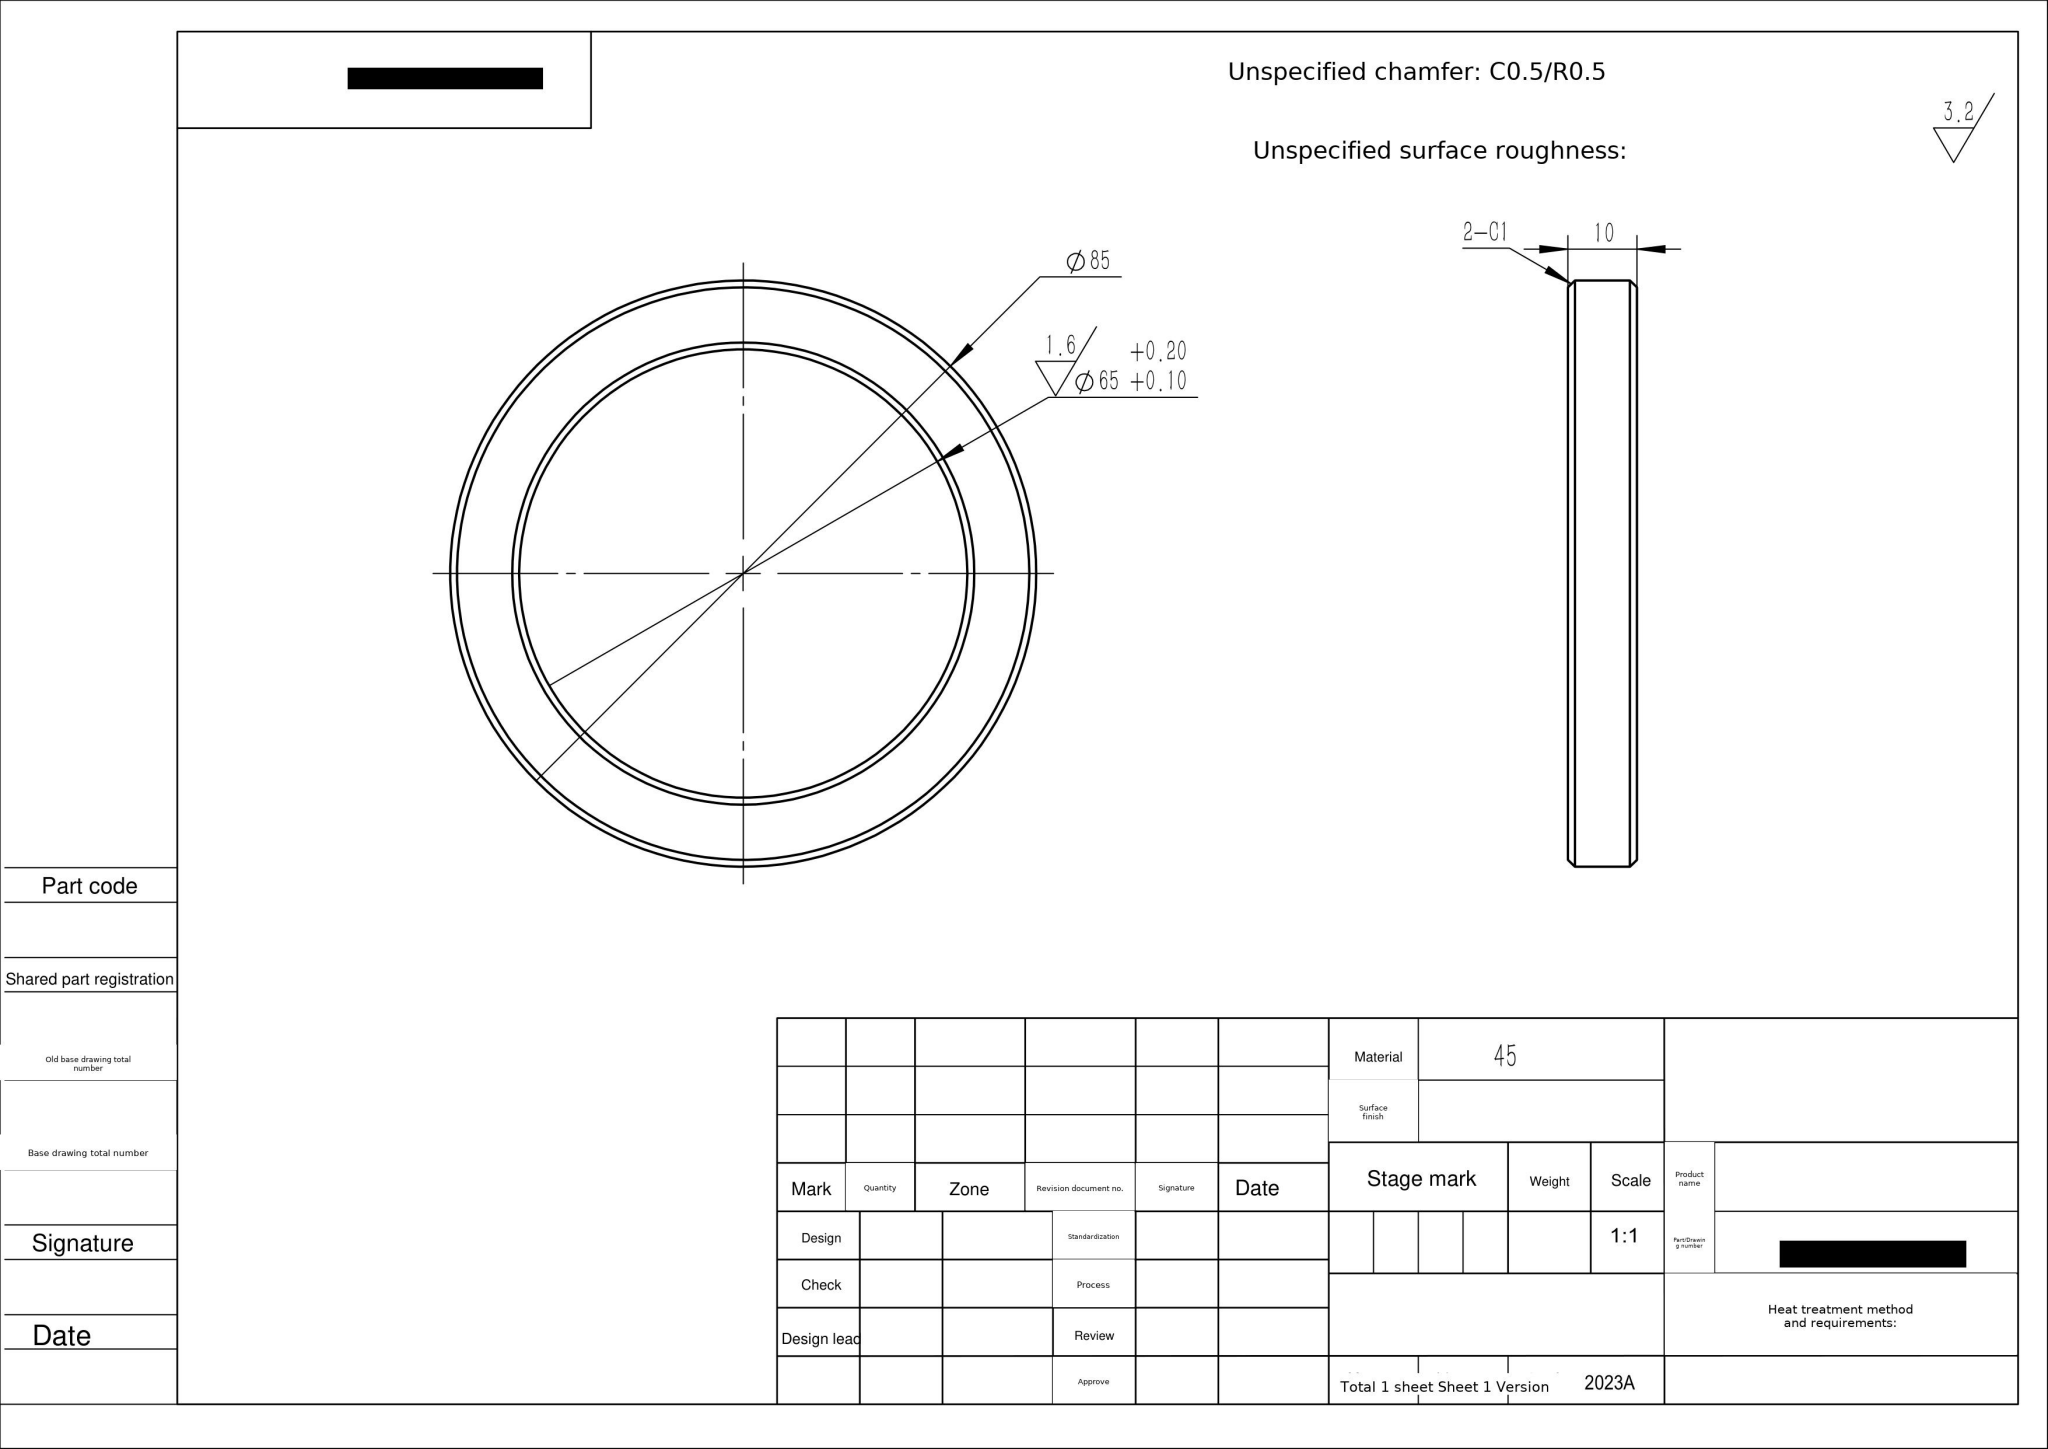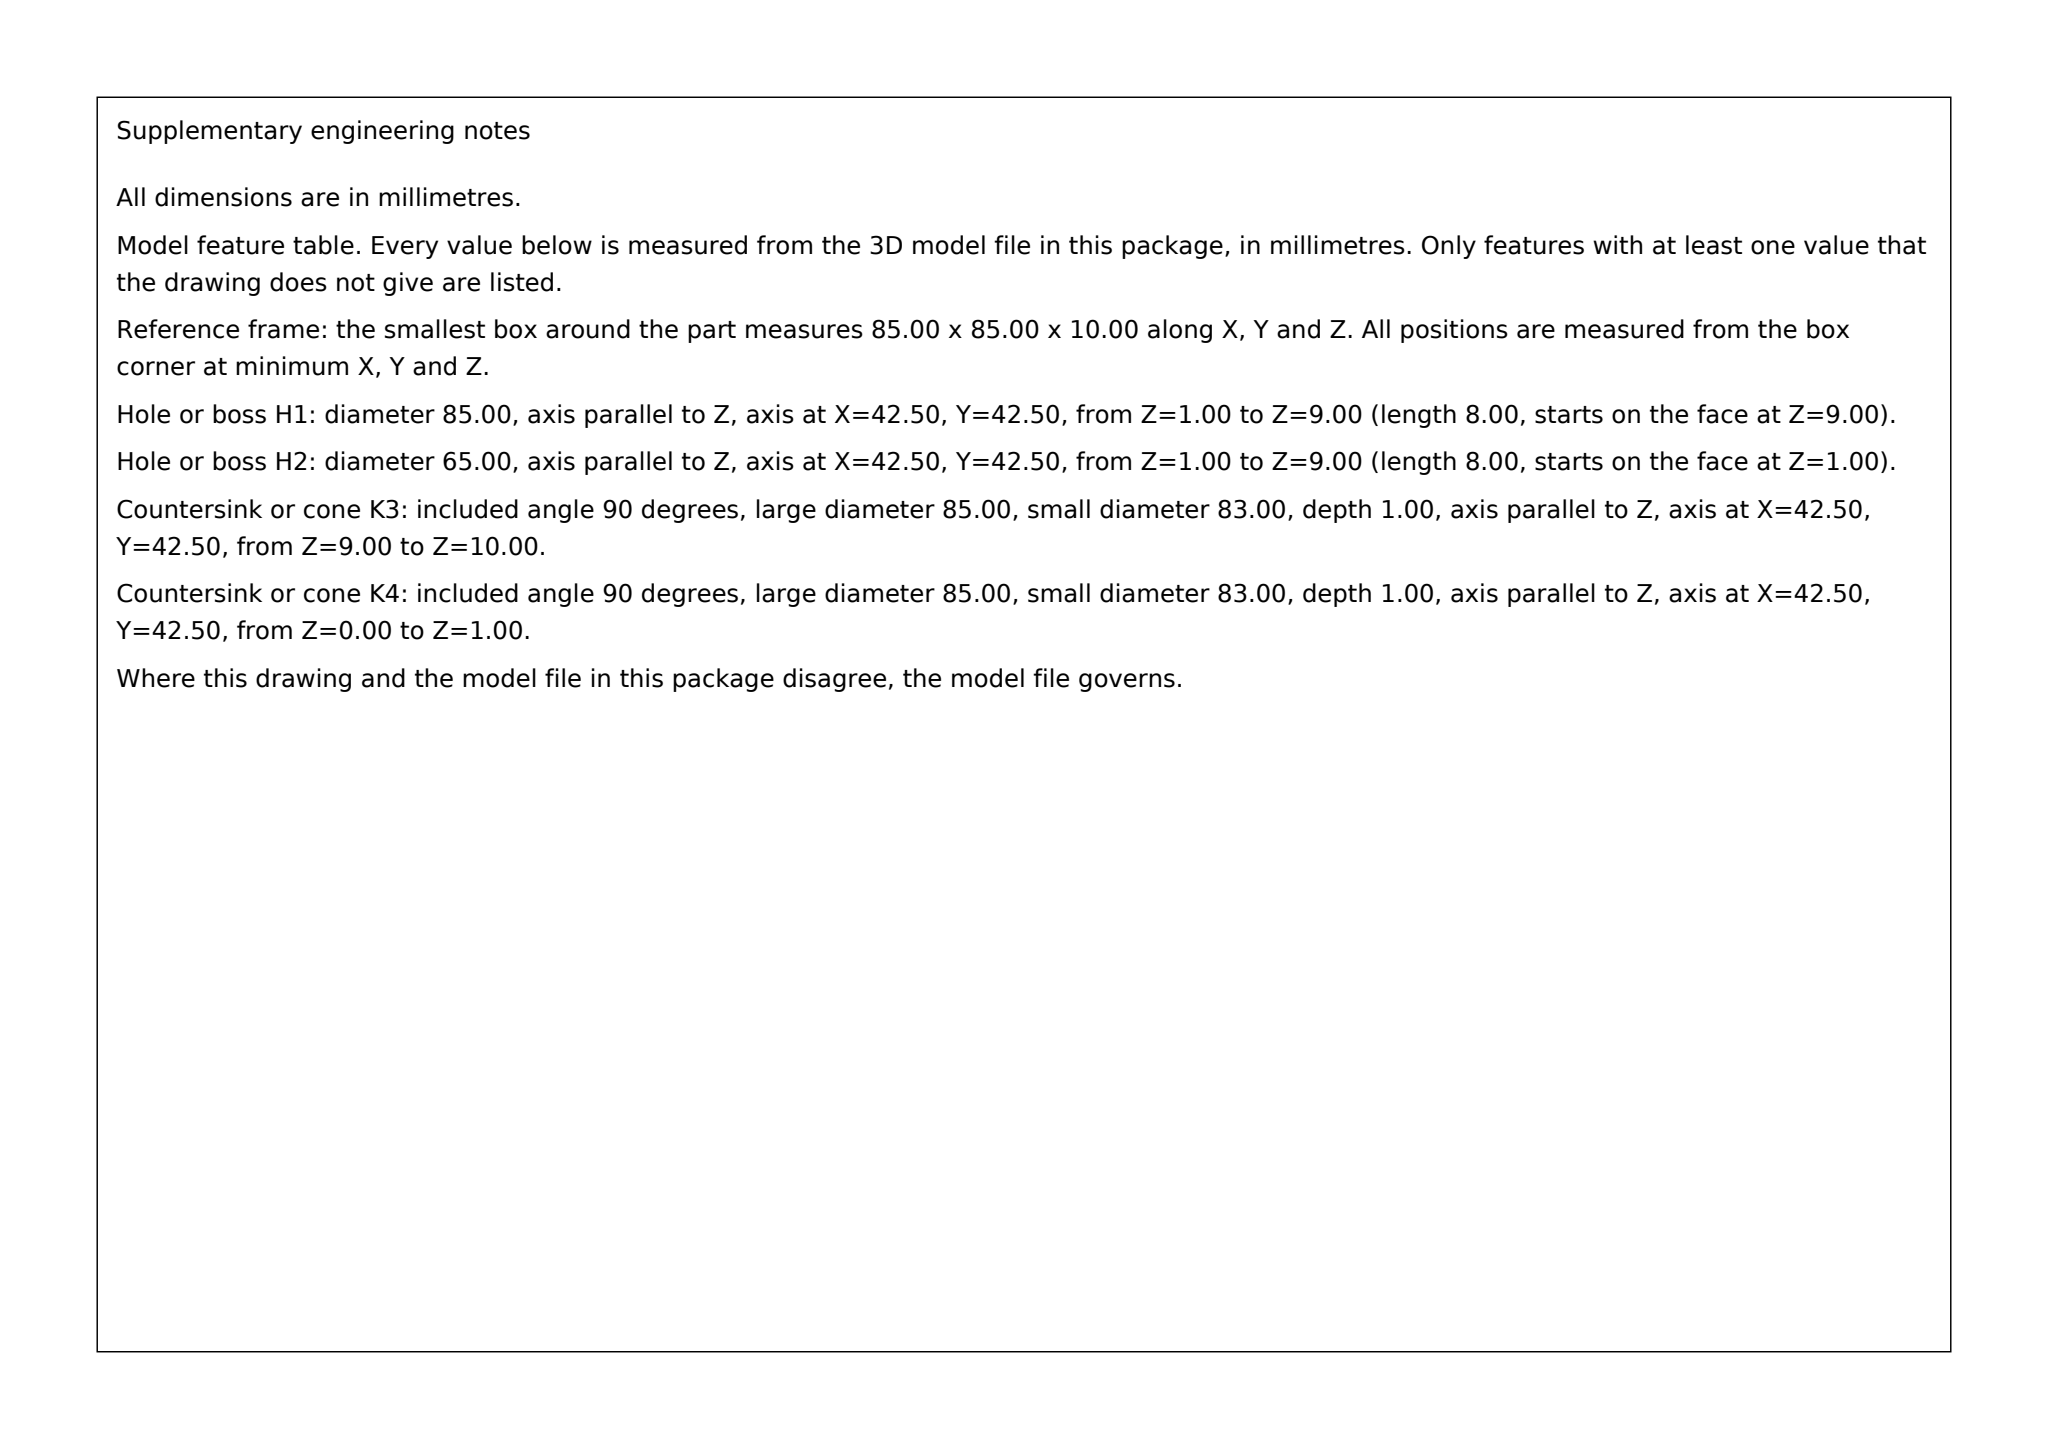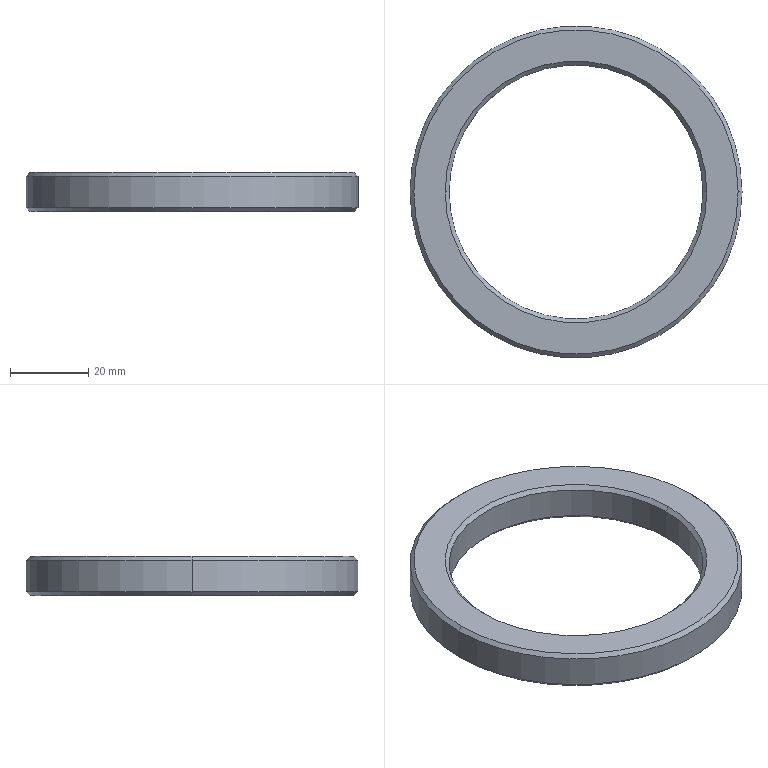Part | SolidWorks | mm | material 45 | 1 solid | 14 faces | box 85 x 85 x 10 mm | volume 23091 mm3 | cone 8 | cylinder 4 | plane 2 | commonest cylinder face diameters 65 x2 85 x2
build123d program:
from build123d import *

# Parameters (mm, degrees)
SKETCH1_R           = 42.5
SKETCH1_R_2         = 32.5
BOSS_EXTRUDE1_DEPTH = 10
CHAMFER1_SIZE       = 1


with BuildPart() as part:
    # Sketch1 → Boss-Extrude1 (new body)
    with BuildSketch(Plane.XY):
        Circle(SKETCH1_R)
        Circle(SKETCH1_R_2, mode=Mode.SUBTRACT)
    extrude(amount=BOSS_EXTRUDE1_DEPTH)

    # Chamfer1
    chamfer1_edges = [part.edges().sort_by_distance(p)[0] for p in [
        (-42.5, 0, 0),
        (-42.5, 0, 10),
        (-32.5, 0, 0),
        (-32.5, 0, 10),
    ]]
    chamfer(chamfer1_edges, length=CHAMFER1_SIZE)


solid = part.part
STEP:
#1=CARTESIAN_POINT('',(41.5,0.,10.));
#2=VERTEX_POINT('',#1);
#3=CARTESIAN_POINT('',(-41.5,0.,10.));
#4=VERTEX_POINT('',#3);
#5=CARTESIAN_POINT('',(0.,0.,10.));
#6=DIRECTION('',(0.,0.,1.));
#7=DIRECTION('',(1.,0.,0.));
#8=AXIS2_PLACEMENT_3D('',#5,#6,#7);
#9=CIRCLE('',#8,41.5);
#10=EDGE_CURVE('',#2,#4,#9,.T.);
#11=ORIENTED_EDGE('',*,*,#10,.F.);
#12=CARTESIAN_POINT('',(42.5,0.,9.));
#13=VERTEX_POINT('',#12);
#14=CARTESIAN_POINT('',(41.5,0.,10.));
#15=DIRECTION('',(0.7071,0.,-0.7071));
#16=VECTOR('',#15,1000.);
#17=LINE('',#14,#16);
#18=EDGE_CURVE('',#2,#13,#17,.T.);
#19=ORIENTED_EDGE('',*,*,#18,.T.);
#20=CARTESIAN_POINT('',(-42.5,0.,9.));
#21=VERTEX_POINT('',#20);
#22=CARTESIAN_POINT('',(0.,0.,9.));
#23=DIRECTION('',(0.,0.,-1.));
#24=DIRECTION('',(1.,0.,0.));
#25=AXIS2_PLACEMENT_3D('',#22,#23,#24);
#26=CIRCLE('',#25,42.5);
#27=EDGE_CURVE('',#21,#13,#26,.T.);
#28=ORIENTED_EDGE('',*,*,#27,.F.);
#29=CARTESIAN_POINT('',(-41.5,0.,10.));
#30=DIRECTION('',(-0.7071,0.,-0.7071));
#31=VECTOR('',#30,1000.);
#32=LINE('',#29,#31);
#33=EDGE_CURVE('',#4,#21,#32,.T.);
#34=ORIENTED_EDGE('',*,*,#33,.F.);
#35=EDGE_LOOP('',(#11,#19,#28,#34));
#36=FACE_OUTER_BOUND('',#35,.T.);
#37=CARTESIAN_POINT('',(0.,0.,10.));
#38=DIRECTION('',(0.,0.,-1.));
#39=DIRECTION('',(-1.,0.,0.));
#40=AXIS2_PLACEMENT_3D('',#37,#38,#39);
#41=CONICAL_SURFACE('',#40,41.5,0.7854);
#42=ADVANCED_FACE('',(#36),#41,.T.);
#43=CARTESIAN_POINT('',(-41.5,0.,0.));
#44=VERTEX_POINT('',#43);
#45=CARTESIAN_POINT('',(41.5,0.,0.));
#46=VERTEX_POINT('',#45);
#47=CARTESIAN_POINT('',(0.,0.,0.));
#48=DIRECTION('',(0.,0.,-1.));
#49=DIRECTION('',(1.,0.,0.));
#50=AXIS2_PLACEMENT_3D('',#47,#48,#49);
#51=CIRCLE('',#50,41.5);
#52=EDGE_CURVE('',#44,#46,#51,.T.);
#53=ORIENTED_EDGE('',*,*,#52,.F.);
#54=CARTESIAN_POINT('',(-42.5,0.,1.));
#55=VERTEX_POINT('',#54);
#56=CARTESIAN_POINT('',(-42.5,0.,1.));
#57=DIRECTION('',(-0.7071,0.,0.7071));
#58=VECTOR('',#57,1000.);
#59=LINE('',#56,#58);
#60=EDGE_CURVE('',#44,#55,#59,.T.);
#61=ORIENTED_EDGE('',*,*,#60,.T.);
#62=CARTESIAN_POINT('',(42.5,0.,1.));
#63=VERTEX_POINT('',#62);
#64=CARTESIAN_POINT('',(0.,0.,1.));
#65=DIRECTION('',(0.,0.,1.));
#66=DIRECTION('',(1.,0.,0.));
#67=AXIS2_PLACEMENT_3D('',#64,#65,#66);
#68=CIRCLE('',#67,42.5);
#69=EDGE_CURVE('',#63,#55,#68,.T.);
#70=ORIENTED_EDGE('',*,*,#69,.F.);
#71=CARTESIAN_POINT('',(42.5,0.,1.));
#72=DIRECTION('',(0.7071,0.,0.7071));
#73=VECTOR('',#72,1000.);
#74=LINE('',#71,#73);
#75=EDGE_CURVE('',#46,#63,#74,.T.);
#76=ORIENTED_EDGE('',*,*,#75,.F.);
#77=EDGE_LOOP('',(#53,#61,#70,#76));
#78=FACE_OUTER_BOUND('',#77,.T.);
#79=CARTESIAN_POINT('',(0.,0.,1.));
#80=DIRECTION('',(0.,0.,1.));
#81=DIRECTION('',(1.,0.,0.));
#82=AXIS2_PLACEMENT_3D('',#79,#80,#81);
#83=CONICAL_SURFACE('',#82,42.5,0.7854);
#84=ADVANCED_FACE('',(#78),#83,.T.);
#85=CARTESIAN_POINT('',(32.5,0.,1.));
#86=VERTEX_POINT('',#85);
#87=CARTESIAN_POINT('',(-32.5,0.,1.));
#88=VERTEX_POINT('',#87);
#89=CARTESIAN_POINT('',(0.,0.,1.));
#90=DIRECTION('',(0.,0.,-1.));
#91=DIRECTION('',(1.,0.,0.));
#92=AXIS2_PLACEMENT_3D('',#89,#90,#91);
#93=CIRCLE('',#92,32.5);
#94=EDGE_CURVE('',#86,#88,#93,.T.);
#95=ORIENTED_EDGE('',*,*,#94,.F.);
#96=CARTESIAN_POINT('',(33.5,0.,0.));
#97=VERTEX_POINT('',#96);
#98=CARTESIAN_POINT('',(33.5,0.,0.));
#99=DIRECTION('',(0.7071,0.,-0.7071));
#100=VECTOR('',#99,1000.);
#101=LINE('',#98,#100);
#102=EDGE_CURVE('',#86,#97,#101,.T.);
#103=ORIENTED_EDGE('',*,*,#102,.T.);
#104=CARTESIAN_POINT('',(-33.5,0.,0.));
#105=VERTEX_POINT('',#104);
#106=CARTESIAN_POINT('',(0.,0.,0.));
#107=DIRECTION('',(0.,0.,1.));
#108=DIRECTION('',(1.,0.,0.));
#109=AXIS2_PLACEMENT_3D('',#106,#107,#108);
#110=CIRCLE('',#109,33.5);
#111=EDGE_CURVE('',#105,#97,#110,.T.);
#112=ORIENTED_EDGE('',*,*,#111,.F.);
#113=CARTESIAN_POINT('',(-33.5,0.,0.));
#114=DIRECTION('',(-0.7071,0.,-0.7071));
#115=VECTOR('',#114,1000.);
#116=LINE('',#113,#115);
#117=EDGE_CURVE('',#88,#105,#116,.T.);
#118=ORIENTED_EDGE('',*,*,#117,.F.);
#119=EDGE_LOOP('',(#95,#103,#112,#118));
#120=FACE_OUTER_BOUND('',#119,.T.);
#121=CARTESIAN_POINT('',(0.,0.,0.));
#122=DIRECTION('',(0.,0.,-1.));
#123=DIRECTION('',(-1.,0.,0.));
#124=AXIS2_PLACEMENT_3D('',#121,#122,#123);
#125=CONICAL_SURFACE('',#124,33.5,0.7854);
#126=ADVANCED_FACE('',(#120),#125,.F.);
#127=CARTESIAN_POINT('',(-32.5,0.,9.));
#128=VERTEX_POINT('',#127);
#129=CARTESIAN_POINT('',(32.5,0.,9.));
#130=VERTEX_POINT('',#129);
#131=CARTESIAN_POINT('',(0.,0.,9.));
#132=DIRECTION('',(0.,0.,1.));
#133=DIRECTION('',(1.,0.,0.));
#134=AXIS2_PLACEMENT_3D('',#131,#132,#133);
#135=CIRCLE('',#134,32.5);
#136=EDGE_CURVE('',#128,#130,#135,.T.);
#137=ORIENTED_EDGE('',*,*,#136,.F.);
#138=CARTESIAN_POINT('',(-33.5,0.,10.));
#139=VERTEX_POINT('',#138);
#140=CARTESIAN_POINT('',(-32.5,0.,9.));
#141=DIRECTION('',(-0.7071,0.,0.7071));
#142=VECTOR('',#141,1000.);
#143=LINE('',#140,#142);
#144=EDGE_CURVE('',#128,#139,#143,.T.);
#145=ORIENTED_EDGE('',*,*,#144,.T.);
#146=CARTESIAN_POINT('',(33.5,0.,10.));
#147=VERTEX_POINT('',#146);
#148=CARTESIAN_POINT('',(0.,0.,10.));
#149=DIRECTION('',(0.,0.,-1.));
#150=DIRECTION('',(1.,0.,0.));
#151=AXIS2_PLACEMENT_3D('',#148,#149,#150);
#152=CIRCLE('',#151,33.5);
#153=EDGE_CURVE('',#147,#139,#152,.T.);
#154=ORIENTED_EDGE('',*,*,#153,.F.);
#155=CARTESIAN_POINT('',(32.5,0.,9.));
#156=DIRECTION('',(0.7071,0.,0.7071));
#157=VECTOR('',#156,1000.);
#158=LINE('',#155,#157);
#159=EDGE_CURVE('',#130,#147,#158,.T.);
#160=ORIENTED_EDGE('',*,*,#159,.F.);
#161=EDGE_LOOP('',(#137,#145,#154,#160));
#162=FACE_OUTER_BOUND('',#161,.T.);
#163=CARTESIAN_POINT('',(0.,0.,9.));
#164=DIRECTION('',(0.,0.,1.));
#165=DIRECTION('',(1.,0.,0.));
#166=AXIS2_PLACEMENT_3D('',#163,#164,#165);
#167=CONICAL_SURFACE('',#166,32.5,0.7854);
#168=ADVANCED_FACE('',(#162),#167,.F.);
#169=ORIENTED_EDGE('',*,*,#136,.T.);
#170=CARTESIAN_POINT('',(32.5,0.,10.));
#171=DIRECTION('',(0.,0.,-1.));
#172=VECTOR('',#171,1000.);
#173=LINE('',#170,#172);
#174=EDGE_CURVE('',#130,#86,#173,.T.);
#175=ORIENTED_EDGE('',*,*,#174,.T.);
#176=ORIENTED_EDGE('',*,*,#94,.T.);
#177=CARTESIAN_POINT('',(-32.5,0.,10.));
#178=DIRECTION('',(0.,0.,-1.));
#179=VECTOR('',#178,1000.);
#180=LINE('',#177,#179);
#181=EDGE_CURVE('',#128,#88,#180,.T.);
#182=ORIENTED_EDGE('',*,*,#181,.F.);
#183=EDGE_LOOP('',(#169,#175,#176,#182));
#184=FACE_OUTER_BOUND('',#183,.T.);
#185=CARTESIAN_POINT('',(0.,0.,10.));
#186=DIRECTION('',(0.,0.,-1.));
#187=DIRECTION('',(-1.,0.,0.));
#188=AXIS2_PLACEMENT_3D('',#185,#186,#187);
#189=CYLINDRICAL_SURFACE('',#188,32.5);
#190=ADVANCED_FACE('',(#184),#189,.F.);
#191=ORIENTED_EDGE('',*,*,#27,.T.);
#192=CARTESIAN_POINT('',(42.5,0.,10.));
#193=DIRECTION('',(0.,0.,-1.));
#194=VECTOR('',#193,1000.);
#195=LINE('',#192,#194);
#196=EDGE_CURVE('',#13,#63,#195,.T.);
#197=ORIENTED_EDGE('',*,*,#196,.T.);
#198=ORIENTED_EDGE('',*,*,#69,.T.);
#199=CARTESIAN_POINT('',(-42.5,0.,10.));
#200=DIRECTION('',(0.,0.,-1.));
#201=VECTOR('',#200,1000.);
#202=LINE('',#199,#201);
#203=EDGE_CURVE('',#21,#55,#202,.T.);
#204=ORIENTED_EDGE('',*,*,#203,.F.);
#205=EDGE_LOOP('',(#191,#197,#198,#204));
#206=FACE_OUTER_BOUND('',#205,.T.);
#207=CARTESIAN_POINT('',(0.,0.,10.));
#208=DIRECTION('',(0.,0.,-1.));
#209=DIRECTION('',(-1.,0.,0.));
#210=AXIS2_PLACEMENT_3D('',#207,#208,#209);
#211=CYLINDRICAL_SURFACE('',#210,42.5);
#212=ADVANCED_FACE('',(#206),#211,.T.);
#213=ORIENTED_EDGE('',*,*,#153,.T.);
#214=CARTESIAN_POINT('',(0.,0.,10.));
#215=DIRECTION('',(0.,0.,-1.));
#216=DIRECTION('',(1.,0.,0.));
#217=AXIS2_PLACEMENT_3D('',#214,#215,#216);
#218=CIRCLE('',#217,33.5);
#219=EDGE_CURVE('',#139,#147,#218,.T.);
#220=ORIENTED_EDGE('',*,*,#219,.T.);
#221=EDGE_LOOP('',(#213,#220));
#222=FACE_BOUND('',#221,.T.);
#223=CARTESIAN_POINT('',(0.,0.,10.));
#224=DIRECTION('',(0.,0.,1.));
#225=DIRECTION('',(1.,0.,0.));
#226=AXIS2_PLACEMENT_3D('',#223,#224,#225);
#227=CIRCLE('',#226,41.5);
#228=EDGE_CURVE('',#4,#2,#227,.T.);
#229=ORIENTED_EDGE('',*,*,#228,.T.);
#230=ORIENTED_EDGE('',*,*,#10,.T.);
#231=EDGE_LOOP('',(#229,#230));
#232=FACE_OUTER_BOUND('',#231,.T.);
#233=CARTESIAN_POINT('',(0.,0.,10.));
#234=DIRECTION('',(0.,0.,1.));
#235=DIRECTION('',(1.,0.,0.));
#236=AXIS2_PLACEMENT_3D('',#233,#234,#235);
#237=PLANE('',#236);
#238=ADVANCED_FACE('',(#222,#232),#237,.T.);
#239=ORIENTED_EDGE('',*,*,#111,.T.);
#240=CARTESIAN_POINT('',(0.,0.,0.));
#241=DIRECTION('',(0.,0.,1.));
#242=DIRECTION('',(1.,0.,0.));
#243=AXIS2_PLACEMENT_3D('',#240,#241,#242);
#244=CIRCLE('',#243,33.5);
#245=EDGE_CURVE('',#97,#105,#244,.T.);
#246=ORIENTED_EDGE('',*,*,#245,.T.);
#247=EDGE_LOOP('',(#239,#246));
#248=FACE_BOUND('',#247,.T.);
#249=CARTESIAN_POINT('',(0.,0.,0.));
#250=DIRECTION('',(0.,0.,-1.));
#251=DIRECTION('',(1.,0.,0.));
#252=AXIS2_PLACEMENT_3D('',#249,#250,#251);
#253=CIRCLE('',#252,41.5);
#254=EDGE_CURVE('',#46,#44,#253,.T.);
#255=ORIENTED_EDGE('',*,*,#254,.T.);
#256=ORIENTED_EDGE('',*,*,#52,.T.);
#257=EDGE_LOOP('',(#255,#256));
#258=FACE_OUTER_BOUND('',#257,.T.);
#259=CARTESIAN_POINT('',(0.,0.,0.));
#260=DIRECTION('',(0.,0.,1.));
#261=DIRECTION('',(1.,0.,0.));
#262=AXIS2_PLACEMENT_3D('',#259,#260,#261);
#263=PLANE('',#262);
#264=ADVANCED_FACE('',(#248,#258),#263,.F.);
#265=ORIENTED_EDGE('',*,*,#196,.F.);
#266=CARTESIAN_POINT('',(0.,0.,9.));
#267=DIRECTION('',(0.,0.,-1.));
#268=DIRECTION('',(1.,0.,0.));
#269=AXIS2_PLACEMENT_3D('',#266,#267,#268);
#270=CIRCLE('',#269,42.5);
#271=EDGE_CURVE('',#13,#21,#270,.T.);
#272=ORIENTED_EDGE('',*,*,#271,.T.);
#273=ORIENTED_EDGE('',*,*,#203,.T.);
#274=CARTESIAN_POINT('',(0.,0.,1.));
#275=DIRECTION('',(0.,0.,1.));
#276=DIRECTION('',(1.,0.,0.));
#277=AXIS2_PLACEMENT_3D('',#274,#275,#276);
#278=CIRCLE('',#277,42.5);
#279=EDGE_CURVE('',#55,#63,#278,.T.);
#280=ORIENTED_EDGE('',*,*,#279,.T.);
#281=EDGE_LOOP('',(#265,#272,#273,#280));
#282=FACE_OUTER_BOUND('',#281,.T.);
#283=CARTESIAN_POINT('',(0.,0.,10.));
#284=DIRECTION('',(0.,0.,-1.));
#285=DIRECTION('',(-1.,0.,0.));
#286=AXIS2_PLACEMENT_3D('',#283,#284,#285);
#287=CYLINDRICAL_SURFACE('',#286,42.5);
#288=ADVANCED_FACE('',(#282),#287,.T.);
#289=ORIENTED_EDGE('',*,*,#174,.F.);
#290=CARTESIAN_POINT('',(0.,0.,9.));
#291=DIRECTION('',(0.,0.,1.));
#292=DIRECTION('',(1.,0.,0.));
#293=AXIS2_PLACEMENT_3D('',#290,#291,#292);
#294=CIRCLE('',#293,32.5);
#295=EDGE_CURVE('',#130,#128,#294,.T.);
#296=ORIENTED_EDGE('',*,*,#295,.T.);
#297=ORIENTED_EDGE('',*,*,#181,.T.);
#298=CARTESIAN_POINT('',(0.,0.,1.));
#299=DIRECTION('',(0.,0.,-1.));
#300=DIRECTION('',(1.,0.,0.));
#301=AXIS2_PLACEMENT_3D('',#298,#299,#300);
#302=CIRCLE('',#301,32.5);
#303=EDGE_CURVE('',#88,#86,#302,.T.);
#304=ORIENTED_EDGE('',*,*,#303,.T.);
#305=EDGE_LOOP('',(#289,#296,#297,#304));
#306=FACE_OUTER_BOUND('',#305,.T.);
#307=CARTESIAN_POINT('',(0.,0.,10.));
#308=DIRECTION('',(0.,0.,-1.));
#309=DIRECTION('',(-1.,0.,0.));
#310=AXIS2_PLACEMENT_3D('',#307,#308,#309);
#311=CYLINDRICAL_SURFACE('',#310,32.5);
#312=ADVANCED_FACE('',(#306),#311,.F.);
#313=ORIENTED_EDGE('',*,*,#144,.F.);
#314=ORIENTED_EDGE('',*,*,#295,.F.);
#315=ORIENTED_EDGE('',*,*,#159,.T.);
#316=ORIENTED_EDGE('',*,*,#219,.F.);
#317=EDGE_LOOP('',(#313,#314,#315,#316));
#318=FACE_OUTER_BOUND('',#317,.T.);
#319=CARTESIAN_POINT('',(0.,0.,9.));
#320=DIRECTION('',(0.,0.,1.));
#321=DIRECTION('',(1.,0.,0.));
#322=AXIS2_PLACEMENT_3D('',#319,#320,#321);
#323=CONICAL_SURFACE('',#322,32.5,0.7854);
#324=ADVANCED_FACE('',(#318),#323,.F.);
#325=ORIENTED_EDGE('',*,*,#102,.F.);
#326=ORIENTED_EDGE('',*,*,#303,.F.);
#327=ORIENTED_EDGE('',*,*,#117,.T.);
#328=ORIENTED_EDGE('',*,*,#245,.F.);
#329=EDGE_LOOP('',(#325,#326,#327,#328));
#330=FACE_OUTER_BOUND('',#329,.T.);
#331=CARTESIAN_POINT('',(0.,0.,0.));
#332=DIRECTION('',(0.,0.,-1.));
#333=DIRECTION('',(-1.,0.,0.));
#334=AXIS2_PLACEMENT_3D('',#331,#332,#333);
#335=CONICAL_SURFACE('',#334,33.5,0.7854);
#336=ADVANCED_FACE('',(#330),#335,.F.);
#337=ORIENTED_EDGE('',*,*,#60,.F.);
#338=ORIENTED_EDGE('',*,*,#254,.F.);
#339=ORIENTED_EDGE('',*,*,#75,.T.);
#340=ORIENTED_EDGE('',*,*,#279,.F.);
#341=EDGE_LOOP('',(#337,#338,#339,#340));
#342=FACE_OUTER_BOUND('',#341,.T.);
#343=CARTESIAN_POINT('',(0.,0.,1.));
#344=DIRECTION('',(0.,0.,1.));
#345=DIRECTION('',(1.,0.,0.));
#346=AXIS2_PLACEMENT_3D('',#343,#344,#345);
#347=CONICAL_SURFACE('',#346,42.5,0.7854);
#348=ADVANCED_FACE('',(#342),#347,.T.);
#349=ORIENTED_EDGE('',*,*,#18,.F.);
#350=ORIENTED_EDGE('',*,*,#228,.F.);
#351=ORIENTED_EDGE('',*,*,#33,.T.);
#352=ORIENTED_EDGE('',*,*,#271,.F.);
#353=EDGE_LOOP('',(#349,#350,#351,#352));
#354=FACE_OUTER_BOUND('',#353,.T.);
#355=CARTESIAN_POINT('',(0.,0.,10.));
#356=DIRECTION('',(0.,0.,-1.));
#357=DIRECTION('',(-1.,0.,0.));
#358=AXIS2_PLACEMENT_3D('',#355,#356,#357);
#359=CONICAL_SURFACE('',#358,41.5,0.7854);
#360=ADVANCED_FACE('',(#354),#359,.T.);
#361=CLOSED_SHELL('',(#42,#84,#126,#168,#190,#212,#238,#264,#288,#312,#324,#336,#348,#360));
#362=MANIFOLD_SOLID_BREP('',#361);
#363=CARTESIAN_POINT('',(0.,0.,0.));
#364=DIRECTION('',(0.,0.,1.));
#365=DIRECTION('',(1.,0.,0.));
#366=AXIS2_PLACEMENT_3D('',#363,#364,#365);
#367=(LENGTH_UNIT()NAMED_UNIT(*)SI_UNIT(.MILLI.,.METRE.));
#368=UNCERTAINTY_MEASURE_WITH_UNIT(LENGTH_MEASURE(0.00001),#367,'','');
#369=(NAMED_UNIT(*)PLANE_ANGLE_UNIT()SI_UNIT($,.RADIAN.));
#370=(NAMED_UNIT(*)SI_UNIT($,.STERADIAN.)SOLID_ANGLE_UNIT());
#371=(GEOMETRIC_REPRESENTATION_CONTEXT(3)GLOBAL_UNCERTAINTY_ASSIGNED_CONTEXT((#368))GLOBAL_UNIT_ASSIGNED_CONTEXT((#367,#369,#370))REPRESENTATION_CONTEXT('',''));
#372=ADVANCED_BREP_SHAPE_REPRESENTATION('',(#362,#366),#371);